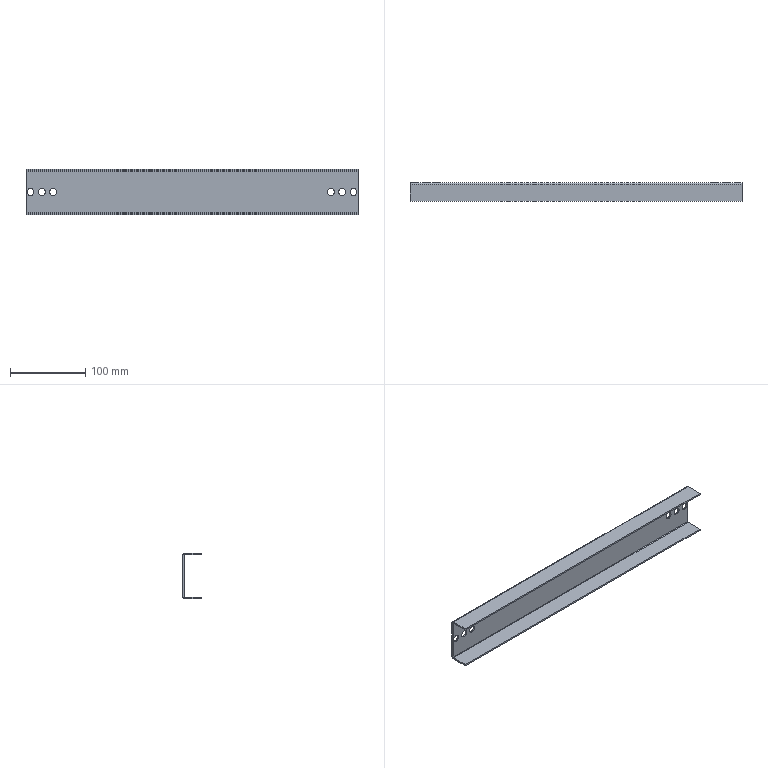Component | SolidWorks | 500CabinetWidthDoorCrossbeamAssembly-1_500CabinetWidthDoorCrossbeam-1 | 1 solid | 34 faces | box 440 x 25 x 60 mm | volume 91170 mm3 | plane 18 | cylinder 16 | commonest cylinder face diameters 9.2 x12 5.473 x2 1.473 x2 | material Plain Carbon Steel
STEP:
#1=COLOUR_RGB('',0.7922,0.8196,0.9333);
#2=FILL_AREA_STYLE_COLOUR('',#1);
#3=FILL_AREA_STYLE('',(#2));
#4=SURFACE_STYLE_FILL_AREA(#3);
#5=SURFACE_SIDE_STYLE('',(#4));
#6=SURFACE_STYLE_USAGE(.BOTH.,#5);
#7=PRESENTATION_STYLE_ASSIGNMENT((#6));
#8=CARTESIAN_POINT('',(-51.435,6.867,86.05));
#9=VERTEX_POINT('',#8);
#10=CARTESIAN_POINT('',(-51.435,6.867,86.412));
#11=VERTEX_POINT('',#10);
#12=CARTESIAN_POINT('',(-51.435,6.867,86.231));
#13=DIRECTION('',(-0.,1.,-0.));
#14=DIRECTION('',(0.,0.,1.));
#15=AXIS2_PLACEMENT_3D('',#12,#13,#14);
#16=CIRCLE('',#15,0.1811);
#17=EDGE_CURVE('',#9,#11,#16,.T.);
#18=ORIENTED_EDGE('',*,*,#17,.F.);
#19=CARTESIAN_POINT('',(-51.435,6.946,86.05));
#20=VERTEX_POINT('',#19);
#21=CARTESIAN_POINT('',(-51.435,6.867,86.05));
#22=DIRECTION('',(-0.,1.,-0.));
#23=VECTOR('',#22,39.37);
#24=LINE('',#21,#23);
#25=EDGE_CURVE('',#9,#20,#24,.T.);
#26=ORIENTED_EDGE('',*,*,#25,.T.);
#27=CARTESIAN_POINT('',(-51.435,6.946,86.412));
#28=VERTEX_POINT('',#27);
#29=CARTESIAN_POINT('',(-51.435,6.946,86.231));
#30=DIRECTION('',(-0.,1.,-0.));
#31=DIRECTION('',(0.,0.,1.));
#32=AXIS2_PLACEMENT_3D('',#29,#30,#31);
#33=CIRCLE('',#32,0.1811);
#34=EDGE_CURVE('',#20,#28,#33,.T.);
#35=ORIENTED_EDGE('',*,*,#34,.T.);
#36=CARTESIAN_POINT('',(-51.435,6.867,86.412));
#37=DIRECTION('',(-0.,1.,-0.));
#38=VECTOR('',#37,39.37);
#39=LINE('',#36,#38);
#40=EDGE_CURVE('',#11,#28,#39,.T.);
#41=ORIENTED_EDGE('',*,*,#40,.F.);
#42=EDGE_LOOP('',(#18,#26,#35,#41));
#43=FACE_OUTER_BOUND('',#42,.T.);
#44=CARTESIAN_POINT('',(-51.435,6.867,86.231));
#45=DIRECTION('',(-0.,1.,-0.));
#46=DIRECTION('',(0.,0.,1.));
#47=AXIS2_PLACEMENT_3D('',#44,#45,#46);
#48=CYLINDRICAL_SURFACE('',#47,0.1811);
#49=ADVANCED_FACE('',(#43),#48,.F.);
#50=CARTESIAN_POINT('',(-52.025,6.867,86.05));
#51=VERTEX_POINT('',#50);
#52=CARTESIAN_POINT('',(-52.025,6.867,86.412));
#53=VERTEX_POINT('',#52);
#54=CARTESIAN_POINT('',(-52.025,6.867,86.231));
#55=DIRECTION('',(-0.,1.,-0.));
#56=DIRECTION('',(0.,0.,1.));
#57=AXIS2_PLACEMENT_3D('',#54,#55,#56);
#58=CIRCLE('',#57,0.1811);
#59=EDGE_CURVE('',#51,#53,#58,.T.);
#60=ORIENTED_EDGE('',*,*,#59,.F.);
#61=CARTESIAN_POINT('',(-52.025,6.946,86.05));
#62=VERTEX_POINT('',#61);
#63=CARTESIAN_POINT('',(-52.025,6.867,86.05));
#64=DIRECTION('',(-0.,1.,-0.));
#65=VECTOR('',#64,39.37);
#66=LINE('',#63,#65);
#67=EDGE_CURVE('',#51,#62,#66,.T.);
#68=ORIENTED_EDGE('',*,*,#67,.T.);
#69=CARTESIAN_POINT('',(-52.025,6.946,86.412));
#70=VERTEX_POINT('',#69);
#71=CARTESIAN_POINT('',(-52.025,6.946,86.231));
#72=DIRECTION('',(-0.,1.,-0.));
#73=DIRECTION('',(0.,0.,1.));
#74=AXIS2_PLACEMENT_3D('',#71,#72,#73);
#75=CIRCLE('',#74,0.1811);
#76=EDGE_CURVE('',#62,#70,#75,.T.);
#77=ORIENTED_EDGE('',*,*,#76,.T.);
#78=CARTESIAN_POINT('',(-52.025,6.867,86.412));
#79=DIRECTION('',(-0.,1.,-0.));
#80=VECTOR('',#79,39.37);
#81=LINE('',#78,#80);
#82=EDGE_CURVE('',#53,#70,#81,.T.);
#83=ORIENTED_EDGE('',*,*,#82,.F.);
#84=EDGE_LOOP('',(#60,#68,#77,#83));
#85=FACE_OUTER_BOUND('',#84,.T.);
#86=CARTESIAN_POINT('',(-52.025,6.867,86.231));
#87=DIRECTION('',(-0.,1.,-0.));
#88=DIRECTION('',(0.,0.,1.));
#89=AXIS2_PLACEMENT_3D('',#86,#87,#88);
#90=CYLINDRICAL_SURFACE('',#89,0.1811);
#91=ADVANCED_FACE('',(#85),#90,.F.);
#92=CARTESIAN_POINT('',(-66.513,6.867,86.05));
#93=VERTEX_POINT('',#92);
#94=CARTESIAN_POINT('',(-66.513,6.867,86.412));
#95=VERTEX_POINT('',#94);
#96=CARTESIAN_POINT('',(-66.513,6.867,86.231));
#97=DIRECTION('',(-0.,1.,-0.));
#98=DIRECTION('',(0.,-0.,-1.));
#99=AXIS2_PLACEMENT_3D('',#96,#97,#98);
#100=CIRCLE('',#99,0.1811);
#101=EDGE_CURVE('',#93,#95,#100,.T.);
#102=ORIENTED_EDGE('',*,*,#101,.F.);
#103=CARTESIAN_POINT('',(-66.513,6.946,86.05));
#104=VERTEX_POINT('',#103);
#105=CARTESIAN_POINT('',(-66.513,6.867,86.05));
#106=DIRECTION('',(-0.,1.,-0.));
#107=VECTOR('',#106,39.37);
#108=LINE('',#105,#107);
#109=EDGE_CURVE('',#93,#104,#108,.T.);
#110=ORIENTED_EDGE('',*,*,#109,.T.);
#111=CARTESIAN_POINT('',(-66.513,6.946,86.412));
#112=VERTEX_POINT('',#111);
#113=CARTESIAN_POINT('',(-66.513,6.946,86.231));
#114=DIRECTION('',(-0.,1.,-0.));
#115=DIRECTION('',(0.,-0.,-1.));
#116=AXIS2_PLACEMENT_3D('',#113,#114,#115);
#117=CIRCLE('',#116,0.1811);
#118=EDGE_CURVE('',#104,#112,#117,.T.);
#119=ORIENTED_EDGE('',*,*,#118,.T.);
#120=CARTESIAN_POINT('',(-66.513,6.867,86.412));
#121=DIRECTION('',(-0.,1.,-0.));
#122=VECTOR('',#121,39.37);
#123=LINE('',#120,#122);
#124=EDGE_CURVE('',#95,#112,#123,.T.);
#125=ORIENTED_EDGE('',*,*,#124,.F.);
#126=EDGE_LOOP('',(#102,#110,#119,#125));
#127=FACE_OUTER_BOUND('',#126,.T.);
#128=CARTESIAN_POINT('',(-66.513,6.867,86.231));
#129=DIRECTION('',(-0.,1.,-0.));
#130=DIRECTION('',(0.,0.,1.));
#131=AXIS2_PLACEMENT_3D('',#128,#129,#130);
#132=CYLINDRICAL_SURFACE('',#131,0.1811);
#133=ADVANCED_FACE('',(#127),#132,.F.);
#134=CARTESIAN_POINT('',(-67.104,6.867,86.05));
#135=VERTEX_POINT('',#134);
#136=CARTESIAN_POINT('',(-67.104,6.867,86.412));
#137=VERTEX_POINT('',#136);
#138=CARTESIAN_POINT('',(-67.104,6.867,86.231));
#139=DIRECTION('',(-0.,1.,-0.));
#140=DIRECTION('',(0.,-0.,-1.));
#141=AXIS2_PLACEMENT_3D('',#138,#139,#140);
#142=CIRCLE('',#141,0.1811);
#143=EDGE_CURVE('',#135,#137,#142,.T.);
#144=ORIENTED_EDGE('',*,*,#143,.F.);
#145=CARTESIAN_POINT('',(-67.104,6.946,86.05));
#146=VERTEX_POINT('',#145);
#147=CARTESIAN_POINT('',(-67.104,6.867,86.05));
#148=DIRECTION('',(-0.,1.,-0.));
#149=VECTOR('',#148,39.37);
#150=LINE('',#147,#149);
#151=EDGE_CURVE('',#135,#146,#150,.T.);
#152=ORIENTED_EDGE('',*,*,#151,.T.);
#153=CARTESIAN_POINT('',(-67.104,6.946,86.412));
#154=VERTEX_POINT('',#153);
#155=CARTESIAN_POINT('',(-67.104,6.946,86.231));
#156=DIRECTION('',(-0.,1.,-0.));
#157=DIRECTION('',(0.,-0.,-1.));
#158=AXIS2_PLACEMENT_3D('',#155,#156,#157);
#159=CIRCLE('',#158,0.1811);
#160=EDGE_CURVE('',#146,#154,#159,.T.);
#161=ORIENTED_EDGE('',*,*,#160,.T.);
#162=CARTESIAN_POINT('',(-67.104,6.867,86.412));
#163=DIRECTION('',(-0.,1.,-0.));
#164=VECTOR('',#163,39.37);
#165=LINE('',#162,#164);
#166=EDGE_CURVE('',#137,#154,#165,.T.);
#167=ORIENTED_EDGE('',*,*,#166,.F.);
#168=EDGE_LOOP('',(#144,#152,#161,#167));
#169=FACE_OUTER_BOUND('',#168,.T.);
#170=CARTESIAN_POINT('',(-67.104,6.867,86.231));
#171=DIRECTION('',(-0.,1.,-0.));
#172=DIRECTION('',(0.,0.,1.));
#173=AXIS2_PLACEMENT_3D('',#170,#171,#172);
#174=CYLINDRICAL_SURFACE('',#173,0.1811);
#175=ADVANCED_FACE('',(#169),#174,.F.);
#176=CARTESIAN_POINT('',(-67.694,6.867,86.05));
#177=VERTEX_POINT('',#176);
#178=CARTESIAN_POINT('',(-67.694,6.867,86.412));
#179=VERTEX_POINT('',#178);
#180=CARTESIAN_POINT('',(-67.694,6.867,86.231));
#181=DIRECTION('',(-0.,1.,-0.));
#182=DIRECTION('',(0.,-0.,-1.));
#183=AXIS2_PLACEMENT_3D('',#180,#181,#182);
#184=CIRCLE('',#183,0.1811);
#185=EDGE_CURVE('',#177,#179,#184,.T.);
#186=ORIENTED_EDGE('',*,*,#185,.F.);
#187=CARTESIAN_POINT('',(-67.694,6.946,86.05));
#188=VERTEX_POINT('',#187);
#189=CARTESIAN_POINT('',(-67.694,6.867,86.05));
#190=DIRECTION('',(-0.,1.,-0.));
#191=VECTOR('',#190,39.37);
#192=LINE('',#189,#191);
#193=EDGE_CURVE('',#177,#188,#192,.T.);
#194=ORIENTED_EDGE('',*,*,#193,.T.);
#195=CARTESIAN_POINT('',(-67.694,6.946,86.412));
#196=VERTEX_POINT('',#195);
#197=CARTESIAN_POINT('',(-67.694,6.946,86.231));
#198=DIRECTION('',(-0.,1.,-0.));
#199=DIRECTION('',(0.,-0.,-1.));
#200=AXIS2_PLACEMENT_3D('',#197,#198,#199);
#201=CIRCLE('',#200,0.1811);
#202=EDGE_CURVE('',#188,#196,#201,.T.);
#203=ORIENTED_EDGE('',*,*,#202,.T.);
#204=CARTESIAN_POINT('',(-67.694,6.867,86.412));
#205=DIRECTION('',(-0.,1.,-0.));
#206=VECTOR('',#205,39.37);
#207=LINE('',#204,#206);
#208=EDGE_CURVE('',#179,#196,#207,.T.);
#209=ORIENTED_EDGE('',*,*,#208,.F.);
#210=EDGE_LOOP('',(#186,#194,#203,#209));
#211=FACE_OUTER_BOUND('',#210,.T.);
#212=CARTESIAN_POINT('',(-67.694,6.867,86.231));
#213=DIRECTION('',(-0.,1.,-0.));
#214=DIRECTION('',(0.,0.,1.));
#215=AXIS2_PLACEMENT_3D('',#212,#213,#214);
#216=CYLINDRICAL_SURFACE('',#215,0.1811);
#217=ADVANCED_FACE('',(#211),#216,.F.);
#218=CARTESIAN_POINT('',(-50.844,6.867,86.05));
#219=VERTEX_POINT('',#218);
#220=CARTESIAN_POINT('',(-50.844,6.867,86.412));
#221=VERTEX_POINT('',#220);
#222=CARTESIAN_POINT('',(-50.844,6.867,86.231));
#223=DIRECTION('',(-0.,1.,-0.));
#224=DIRECTION('',(0.,0.,1.));
#225=AXIS2_PLACEMENT_3D('',#222,#223,#224);
#226=CIRCLE('',#225,0.1811);
#227=EDGE_CURVE('',#219,#221,#226,.T.);
#228=ORIENTED_EDGE('',*,*,#227,.F.);
#229=CARTESIAN_POINT('',(-50.844,6.946,86.05));
#230=VERTEX_POINT('',#229);
#231=CARTESIAN_POINT('',(-50.844,6.867,86.05));
#232=DIRECTION('',(-0.,1.,-0.));
#233=VECTOR('',#232,39.37);
#234=LINE('',#231,#233);
#235=EDGE_CURVE('',#219,#230,#234,.T.);
#236=ORIENTED_EDGE('',*,*,#235,.T.);
#237=CARTESIAN_POINT('',(-50.844,6.946,86.412));
#238=VERTEX_POINT('',#237);
#239=CARTESIAN_POINT('',(-50.844,6.946,86.231));
#240=DIRECTION('',(-0.,1.,-0.));
#241=DIRECTION('',(0.,0.,1.));
#242=AXIS2_PLACEMENT_3D('',#239,#240,#241);
#243=CIRCLE('',#242,0.1811);
#244=EDGE_CURVE('',#230,#238,#243,.T.);
#245=ORIENTED_EDGE('',*,*,#244,.T.);
#246=CARTESIAN_POINT('',(-50.844,6.867,86.412));
#247=DIRECTION('',(-0.,1.,-0.));
#248=VECTOR('',#247,39.37);
#249=LINE('',#246,#248);
#250=EDGE_CURVE('',#221,#238,#249,.T.);
#251=ORIENTED_EDGE('',*,*,#250,.F.);
#252=EDGE_LOOP('',(#228,#236,#245,#251));
#253=FACE_OUTER_BOUND('',#252,.T.);
#254=CARTESIAN_POINT('',(-50.844,6.867,86.231));
#255=DIRECTION('',(-0.,1.,-0.));
#256=DIRECTION('',(0.,0.,1.));
#257=AXIS2_PLACEMENT_3D('',#254,#255,#256);
#258=CYLINDRICAL_SURFACE('',#257,0.1811);
#259=ADVANCED_FACE('',(#253),#258,.F.);
#260=CARTESIAN_POINT('',(-50.608,6.946,87.304));
#261=VERTEX_POINT('',#260);
#262=CARTESIAN_POINT('',(-50.608,6.867,87.304));
#263=VERTEX_POINT('',#262);
#264=CARTESIAN_POINT('',(-50.608,6.946,87.304));
#265=DIRECTION('',(0.,-1.,0.));
#266=VECTOR('',#265,39.37);
#267=LINE('',#264,#266);
#268=EDGE_CURVE('',#261,#263,#267,.T.);
#269=ORIENTED_EDGE('',*,*,#268,.F.);
#270=CARTESIAN_POINT('',(-50.608,6.838,87.412));
#271=VERTEX_POINT('',#270);
#272=CARTESIAN_POINT('',(-50.608,6.838,87.304));
#273=DIRECTION('',(-1.,-0.,-0.));
#274=DIRECTION('',(0.,0.,1.));
#275=AXIS2_PLACEMENT_3D('',#272,#273,#274);
#276=CIRCLE('',#275,0.1077);
#277=EDGE_CURVE('',#271,#261,#276,.T.);
#278=ORIENTED_EDGE('',*,*,#277,.F.);
#279=CARTESIAN_POINT('',(-50.608,6.838,87.333));
#280=VERTEX_POINT('',#279);
#281=CARTESIAN_POINT('',(-50.608,6.838,87.333));
#282=DIRECTION('',(-0.,0.,1.));
#283=VECTOR('',#282,39.37);
#284=LINE('',#281,#283);
#285=EDGE_CURVE('',#280,#271,#284,.T.);
#286=ORIENTED_EDGE('',*,*,#285,.F.);
#287=CARTESIAN_POINT('',(-50.608,6.838,87.304));
#288=DIRECTION('',(-1.,-0.,-0.));
#289=DIRECTION('',(0.,-1.,0.));
#290=AXIS2_PLACEMENT_3D('',#287,#288,#289);
#291=CIRCLE('',#290,0.029);
#292=EDGE_CURVE('',#280,#263,#291,.T.);
#293=ORIENTED_EDGE('',*,*,#292,.T.);
#294=EDGE_LOOP('',(#269,#278,#286,#293));
#295=FACE_OUTER_BOUND('',#294,.T.);
#296=CARTESIAN_POINT('',(-50.608,6.946,87.304));
#297=DIRECTION('',(1.,0.,0.));
#298=DIRECTION('',(-0.,0.,1.));
#299=AXIS2_PLACEMENT_3D('',#296,#297,#298);
#300=PLANE('',#299);
#301=ADVANCED_FACE('',(#295),#300,.T.);
#302=CARTESIAN_POINT('',(-50.608,6.946,85.158));
#303=VERTEX_POINT('',#302);
#304=CARTESIAN_POINT('',(-50.608,6.946,87.412));
#305=DIRECTION('',(0.,-0.,-1.));
#306=VECTOR('',#305,39.37);
#307=LINE('',#304,#306);
#308=EDGE_CURVE('',#261,#303,#307,.T.);
#309=ORIENTED_EDGE('',*,*,#308,.F.);
#310=ORIENTED_EDGE('',*,*,#268,.T.);
#311=CARTESIAN_POINT('',(-50.608,6.867,85.158));
#312=VERTEX_POINT('',#311);
#313=CARTESIAN_POINT('',(-50.608,6.867,87.412));
#314=DIRECTION('',(0.,-0.,-1.));
#315=VECTOR('',#314,39.37);
#316=LINE('',#313,#315);
#317=EDGE_CURVE('',#263,#312,#316,.T.);
#318=ORIENTED_EDGE('',*,*,#317,.T.);
#319=CARTESIAN_POINT('',(-50.608,6.867,85.158));
#320=DIRECTION('',(-0.,1.,-0.));
#321=VECTOR('',#320,39.37);
#322=LINE('',#319,#321);
#323=EDGE_CURVE('',#312,#303,#322,.T.);
#324=ORIENTED_EDGE('',*,*,#323,.T.);
#325=EDGE_LOOP('',(#309,#310,#318,#324));
#326=FACE_OUTER_BOUND('',#325,.T.);
#327=CARTESIAN_POINT('',(-50.608,6.838,87.333));
#328=DIRECTION('',(1.,0.,0.));
#329=DIRECTION('',(-0.,0.,1.));
#330=AXIS2_PLACEMENT_3D('',#327,#328,#329);
#331=PLANE('',#330);
#332=ADVANCED_FACE('',(#326),#331,.T.);
#333=CARTESIAN_POINT('',(-67.931,6.838,87.412));
#334=VERTEX_POINT('',#333);
#335=CARTESIAN_POINT('',(-67.931,6.838,87.333));
#336=VERTEX_POINT('',#335);
#337=CARTESIAN_POINT('',(-67.931,6.838,87.412));
#338=DIRECTION('',(0.,-0.,-1.));
#339=VECTOR('',#338,39.37);
#340=LINE('',#337,#339);
#341=EDGE_CURVE('',#334,#336,#340,.T.);
#342=ORIENTED_EDGE('',*,*,#341,.F.);
#343=CARTESIAN_POINT('',(-67.931,6.946,87.304));
#344=VERTEX_POINT('',#343);
#345=CARTESIAN_POINT('',(-67.931,6.838,87.304));
#346=DIRECTION('',(-1.,-0.,-0.));
#347=DIRECTION('',(0.,0.,1.));
#348=AXIS2_PLACEMENT_3D('',#345,#346,#347);
#349=CIRCLE('',#348,0.1077);
#350=EDGE_CURVE('',#334,#344,#349,.T.);
#351=ORIENTED_EDGE('',*,*,#350,.T.);
#352=CARTESIAN_POINT('',(-67.931,6.867,87.304));
#353=VERTEX_POINT('',#352);
#354=CARTESIAN_POINT('',(-67.931,6.867,87.304));
#355=DIRECTION('',(-0.,1.,-0.));
#356=VECTOR('',#355,39.37);
#357=LINE('',#354,#356);
#358=EDGE_CURVE('',#353,#344,#357,.T.);
#359=ORIENTED_EDGE('',*,*,#358,.F.);
#360=CARTESIAN_POINT('',(-67.931,6.838,87.304));
#361=DIRECTION('',(-1.,-0.,-0.));
#362=DIRECTION('',(0.,-1.,0.));
#363=AXIS2_PLACEMENT_3D('',#360,#361,#362);
#364=CIRCLE('',#363,0.029);
#365=EDGE_CURVE('',#336,#353,#364,.T.);
#366=ORIENTED_EDGE('',*,*,#365,.F.);
#367=EDGE_LOOP('',(#342,#351,#359,#366));
#368=FACE_OUTER_BOUND('',#367,.T.);
#369=CARTESIAN_POINT('',(-67.931,6.838,87.412));
#370=DIRECTION('',(-1.,-0.,-0.));
#371=DIRECTION('',(0.,-0.,-1.));
#372=AXIS2_PLACEMENT_3D('',#369,#370,#371);
#373=PLANE('',#372);
#374=ADVANCED_FACE('',(#368),#373,.T.);
#375=CARTESIAN_POINT('',(-67.931,5.961,87.412));
#376=VERTEX_POINT('',#375);
#377=CARTESIAN_POINT('',(-67.931,5.961,87.412));
#378=DIRECTION('',(-0.,1.,-0.));
#379=VECTOR('',#378,39.37);
#380=LINE('',#377,#379);
#381=EDGE_CURVE('',#376,#334,#380,.T.);
#382=ORIENTED_EDGE('',*,*,#381,.T.);
#383=ORIENTED_EDGE('',*,*,#341,.T.);
#384=CARTESIAN_POINT('',(-67.931,5.961,87.333));
#385=VERTEX_POINT('',#384);
#386=CARTESIAN_POINT('',(-67.931,5.961,87.333));
#387=DIRECTION('',(-0.,1.,-0.));
#388=VECTOR('',#387,39.37);
#389=LINE('',#386,#388);
#390=EDGE_CURVE('',#385,#336,#389,.T.);
#391=ORIENTED_EDGE('',*,*,#390,.F.);
#392=CARTESIAN_POINT('',(-67.931,5.961,87.333));
#393=DIRECTION('',(-0.,0.,1.));
#394=VECTOR('',#393,39.37);
#395=LINE('',#392,#394);
#396=EDGE_CURVE('',#385,#376,#395,.T.);
#397=ORIENTED_EDGE('',*,*,#396,.T.);
#398=EDGE_LOOP('',(#382,#383,#391,#397));
#399=FACE_OUTER_BOUND('',#398,.T.);
#400=CARTESIAN_POINT('',(-67.931,6.867,87.304));
#401=DIRECTION('',(-1.,-0.,-0.));
#402=DIRECTION('',(0.,-0.,-1.));
#403=AXIS2_PLACEMENT_3D('',#400,#401,#402);
#404=PLANE('',#403);
#405=ADVANCED_FACE('',(#399),#404,.T.);
#406=CARTESIAN_POINT('',(-50.608,6.838,85.05));
#407=VERTEX_POINT('',#406);
#408=CARTESIAN_POINT('',(-50.608,6.838,85.129));
#409=VERTEX_POINT('',#408);
#410=CARTESIAN_POINT('',(-50.608,6.838,85.05));
#411=DIRECTION('',(-0.,0.,1.));
#412=VECTOR('',#411,39.37);
#413=LINE('',#410,#412);
#414=EDGE_CURVE('',#407,#409,#413,.T.);
#415=ORIENTED_EDGE('',*,*,#414,.F.);
#416=CARTESIAN_POINT('',(-50.608,6.838,85.158));
#417=DIRECTION('',(-1.,-0.,-0.));
#418=DIRECTION('',(0.,0.,1.));
#419=AXIS2_PLACEMENT_3D('',#416,#417,#418);
#420=CIRCLE('',#419,0.1077);
#421=EDGE_CURVE('',#303,#407,#420,.T.);
#422=ORIENTED_EDGE('',*,*,#421,.F.);
#423=ORIENTED_EDGE('',*,*,#323,.F.);
#424=CARTESIAN_POINT('',(-50.608,6.838,85.158));
#425=DIRECTION('',(-1.,-0.,-0.));
#426=DIRECTION('',(0.,-1.,0.));
#427=AXIS2_PLACEMENT_3D('',#424,#425,#426);
#428=CIRCLE('',#427,0.029);
#429=EDGE_CURVE('',#312,#409,#428,.T.);
#430=ORIENTED_EDGE('',*,*,#429,.T.);
#431=EDGE_LOOP('',(#415,#422,#423,#430));
#432=FACE_OUTER_BOUND('',#431,.T.);
#433=CARTESIAN_POINT('',(-50.608,6.838,85.05));
#434=DIRECTION('',(1.,0.,0.));
#435=DIRECTION('',(-0.,0.,1.));
#436=AXIS2_PLACEMENT_3D('',#433,#434,#435);
#437=PLANE('',#436);
#438=ADVANCED_FACE('',(#432),#437,.T.);
#439=CARTESIAN_POINT('',(-50.608,5.961,85.05));
#440=VERTEX_POINT('',#439);
#441=CARTESIAN_POINT('',(-50.608,6.946,85.05));
#442=DIRECTION('',(0.,-1.,0.));
#443=VECTOR('',#442,39.37);
#444=LINE('',#441,#443);
#445=EDGE_CURVE('',#407,#440,#444,.T.);
#446=ORIENTED_EDGE('',*,*,#445,.F.);
#447=ORIENTED_EDGE('',*,*,#414,.T.);
#448=CARTESIAN_POINT('',(-50.608,5.961,85.129));
#449=VERTEX_POINT('',#448);
#450=CARTESIAN_POINT('',(-50.608,6.946,85.129));
#451=DIRECTION('',(0.,-1.,0.));
#452=VECTOR('',#451,39.37);
#453=LINE('',#450,#452);
#454=EDGE_CURVE('',#409,#449,#453,.T.);
#455=ORIENTED_EDGE('',*,*,#454,.T.);
#456=CARTESIAN_POINT('',(-50.608,5.961,85.05));
#457=DIRECTION('',(-0.,0.,1.));
#458=VECTOR('',#457,39.37);
#459=LINE('',#456,#458);
#460=EDGE_CURVE('',#440,#449,#459,.T.);
#461=ORIENTED_EDGE('',*,*,#460,.F.);
#462=EDGE_LOOP('',(#446,#447,#455,#461));
#463=FACE_OUTER_BOUND('',#462,.T.);
#464=CARTESIAN_POINT('',(-50.608,6.867,85.158));
#465=DIRECTION('',(1.,0.,0.));
#466=DIRECTION('',(-0.,0.,1.));
#467=AXIS2_PLACEMENT_3D('',#464,#465,#466);
#468=PLANE('',#467);
#469=ADVANCED_FACE('',(#463),#468,.T.);
#470=CARTESIAN_POINT('',(-67.931,6.946,85.158));
#471=VERTEX_POINT('',#470);
#472=CARTESIAN_POINT('',(-67.931,6.867,85.158));
#473=VERTEX_POINT('',#472);
#474=CARTESIAN_POINT('',(-67.931,6.946,85.158));
#475=DIRECTION('',(0.,-1.,0.));
#476=VECTOR('',#475,39.37);
#477=LINE('',#474,#476);
#478=EDGE_CURVE('',#471,#473,#477,.T.);
#479=ORIENTED_EDGE('',*,*,#478,.F.);
#480=CARTESIAN_POINT('',(-67.931,6.838,85.05));
#481=VERTEX_POINT('',#480);
#482=CARTESIAN_POINT('',(-67.931,6.838,85.158));
#483=DIRECTION('',(-1.,-0.,-0.));
#484=DIRECTION('',(0.,0.,1.));
#485=AXIS2_PLACEMENT_3D('',#482,#483,#484);
#486=CIRCLE('',#485,0.1077);
#487=EDGE_CURVE('',#471,#481,#486,.T.);
#488=ORIENTED_EDGE('',*,*,#487,.T.);
#489=CARTESIAN_POINT('',(-67.931,6.838,85.129));
#490=VERTEX_POINT('',#489);
#491=CARTESIAN_POINT('',(-67.931,6.838,85.129));
#492=DIRECTION('',(0.,-0.,-1.));
#493=VECTOR('',#492,39.37);
#494=LINE('',#491,#493);
#495=EDGE_CURVE('',#490,#481,#494,.T.);
#496=ORIENTED_EDGE('',*,*,#495,.F.);
#497=CARTESIAN_POINT('',(-67.931,6.838,85.158));
#498=DIRECTION('',(-1.,-0.,-0.));
#499=DIRECTION('',(0.,-1.,0.));
#500=AXIS2_PLACEMENT_3D('',#497,#498,#499);
#501=CIRCLE('',#500,0.029);
#502=EDGE_CURVE('',#473,#490,#501,.T.);
#503=ORIENTED_EDGE('',*,*,#502,.F.);
#504=EDGE_LOOP('',(#479,#488,#496,#503));
#505=FACE_OUTER_BOUND('',#504,.T.);
#506=CARTESIAN_POINT('',(-67.931,6.946,85.158));
#507=DIRECTION('',(-1.,-0.,-0.));
#508=DIRECTION('',(0.,-0.,-1.));
#509=AXIS2_PLACEMENT_3D('',#506,#507,#508);
#510=PLANE('',#509);
#511=ADVANCED_FACE('',(#505),#510,.T.);
#512=CARTESIAN_POINT('',(-67.931,6.946,87.412));
#513=DIRECTION('',(0.,-0.,-1.));
#514=VECTOR('',#513,39.37);
#515=LINE('',#512,#514);
#516=EDGE_CURVE('',#344,#471,#515,.T.);
#517=ORIENTED_EDGE('',*,*,#516,.T.);
#518=ORIENTED_EDGE('',*,*,#478,.T.);
#519=CARTESIAN_POINT('',(-67.931,6.867,87.412));
#520=DIRECTION('',(0.,-0.,-1.));
#521=VECTOR('',#520,39.37);
#522=LINE('',#519,#521);
#523=EDGE_CURVE('',#353,#473,#522,.T.);
#524=ORIENTED_EDGE('',*,*,#523,.F.);
#525=ORIENTED_EDGE('',*,*,#358,.T.);
#526=EDGE_LOOP('',(#517,#518,#524,#525));
#527=FACE_OUTER_BOUND('',#526,.T.);
#528=CARTESIAN_POINT('',(-67.931,6.838,85.129));
#529=DIRECTION('',(-1.,-0.,-0.));
#530=DIRECTION('',(0.,-0.,-1.));
#531=AXIS2_PLACEMENT_3D('',#528,#529,#530);
#532=PLANE('',#531);
#533=ADVANCED_FACE('',(#527),#532,.T.);
#534=CARTESIAN_POINT('',(-67.931,5.961,85.129));
#535=VERTEX_POINT('',#534);
#536=CARTESIAN_POINT('',(-67.931,6.946,85.129));
#537=DIRECTION('',(0.,-1.,0.));
#538=VECTOR('',#537,39.37);
#539=LINE('',#536,#538);
#540=EDGE_CURVE('',#490,#535,#539,.T.);
#541=ORIENTED_EDGE('',*,*,#540,.T.);
#542=CARTESIAN_POINT('',(-50.608,5.961,85.129));
#543=DIRECTION('',(-1.,-0.,-0.));
#544=VECTOR('',#543,39.37);
#545=LINE('',#542,#544);
#546=EDGE_CURVE('',#449,#535,#545,.T.);
#547=ORIENTED_EDGE('',*,*,#546,.F.);
#548=ORIENTED_EDGE('',*,*,#454,.F.);
#549=CARTESIAN_POINT('',(-50.608,6.838,85.129));
#550=DIRECTION('',(-1.,-0.,-0.));
#551=VECTOR('',#550,39.37);
#552=LINE('',#549,#551);
#553=EDGE_CURVE('',#409,#490,#552,.T.);
#554=ORIENTED_EDGE('',*,*,#553,.T.);
#555=EDGE_LOOP('',(#541,#547,#548,#554));
#556=FACE_OUTER_BOUND('',#555,.T.);
#557=CARTESIAN_POINT('',(-50.608,6.946,85.129));
#558=DIRECTION('',(0.,-0.,-1.));
#559=DIRECTION('',(-0.,1.,-0.));
#560=AXIS2_PLACEMENT_3D('',#557,#558,#559);
#561=PLANE('',#560);
#562=ADVANCED_FACE('',(#556),#561,.F.);
#563=CARTESIAN_POINT('',(-67.931,5.961,85.05));
#564=VERTEX_POINT('',#563);
#565=CARTESIAN_POINT('',(-67.931,5.961,85.05));
#566=DIRECTION('',(-0.,0.,1.));
#567=VECTOR('',#566,39.37);
#568=LINE('',#565,#567);
#569=EDGE_CURVE('',#564,#535,#568,.T.);
#570=ORIENTED_EDGE('',*,*,#569,.F.);
#571=CARTESIAN_POINT('',(-50.608,5.961,85.05));
#572=DIRECTION('',(-1.,-0.,-0.));
#573=VECTOR('',#572,39.37);
#574=LINE('',#571,#573);
#575=EDGE_CURVE('',#440,#564,#574,.T.);
#576=ORIENTED_EDGE('',*,*,#575,.F.);
#577=ORIENTED_EDGE('',*,*,#460,.T.);
#578=ORIENTED_EDGE('',*,*,#546,.T.);
#579=EDGE_LOOP('',(#570,#576,#577,#578));
#580=FACE_OUTER_BOUND('',#579,.T.);
#581=CARTESIAN_POINT('',(-50.608,5.961,85.05));
#582=DIRECTION('',(0.,-1.,0.));
#583=DIRECTION('',(0.,-0.,-1.));
#584=AXIS2_PLACEMENT_3D('',#581,#582,#583);
#585=PLANE('',#584);
#586=ADVANCED_FACE('',(#580),#585,.T.);
#587=CARTESIAN_POINT('',(-67.931,6.946,85.05));
#588=DIRECTION('',(0.,-1.,0.));
#589=VECTOR('',#588,39.37);
#590=LINE('',#587,#589);
#591=EDGE_CURVE('',#481,#564,#590,.T.);
#592=ORIENTED_EDGE('',*,*,#591,.F.);
#593=CARTESIAN_POINT('',(-50.608,6.838,85.05));
#594=DIRECTION('',(-1.,-0.,-0.));
#595=VECTOR('',#594,39.37);
#596=LINE('',#593,#595);
#597=EDGE_CURVE('',#407,#481,#596,.T.);
#598=ORIENTED_EDGE('',*,*,#597,.F.);
#599=ORIENTED_EDGE('',*,*,#445,.T.);
#600=ORIENTED_EDGE('',*,*,#575,.T.);
#601=EDGE_LOOP('',(#592,#598,#599,#600));
#602=FACE_OUTER_BOUND('',#601,.T.);
#603=CARTESIAN_POINT('',(-50.608,6.946,85.05));
#604=DIRECTION('',(0.,-0.,-1.));
#605=DIRECTION('',(-0.,1.,-0.));
#606=AXIS2_PLACEMENT_3D('',#603,#604,#605);
#607=PLANE('',#606);
#608=ADVANCED_FACE('',(#602),#607,.T.);
#609=ORIENTED_EDGE('',*,*,#487,.F.);
#610=CARTESIAN_POINT('',(-50.608,6.946,85.158));
#611=DIRECTION('',(-1.,-0.,-0.));
#612=VECTOR('',#611,39.37);
#613=LINE('',#610,#612);
#614=EDGE_CURVE('',#303,#471,#613,.T.);
#615=ORIENTED_EDGE('',*,*,#614,.F.);
#616=ORIENTED_EDGE('',*,*,#421,.T.);
#617=ORIENTED_EDGE('',*,*,#597,.T.);
#618=EDGE_LOOP('',(#609,#615,#616,#617));
#619=FACE_OUTER_BOUND('',#618,.T.);
#620=CARTESIAN_POINT('',(-50.608,6.838,85.158));
#621=DIRECTION('',(-1.,-0.,-0.));
#622=DIRECTION('',(0.,-0.,-1.));
#623=AXIS2_PLACEMENT_3D('',#620,#621,#622);
#624=CYLINDRICAL_SURFACE('',#623,0.1077);
#625=ADVANCED_FACE('',(#619),#624,.T.);
#626=CARTESIAN_POINT('',(-51.435,6.946,86.231));
#627=DIRECTION('',(-0.,1.,-0.));
#628=DIRECTION('',(0.,0.,1.));
#629=AXIS2_PLACEMENT_3D('',#626,#627,#628);
#630=CIRCLE('',#629,0.1811);
#631=EDGE_CURVE('',#28,#20,#630,.T.);
#632=ORIENTED_EDGE('',*,*,#631,.F.);
#633=ORIENTED_EDGE('',*,*,#34,.F.);
#634=EDGE_LOOP('',(#632,#633));
#635=FACE_BOUND('',#634,.T.);
#636=CARTESIAN_POINT('',(-52.025,6.946,86.231));
#637=DIRECTION('',(-0.,1.,-0.));
#638=DIRECTION('',(0.,0.,1.));
#639=AXIS2_PLACEMENT_3D('',#636,#637,#638);
#640=CIRCLE('',#639,0.1811);
#641=EDGE_CURVE('',#70,#62,#640,.T.);
#642=ORIENTED_EDGE('',*,*,#641,.F.);
#643=ORIENTED_EDGE('',*,*,#76,.F.);
#644=EDGE_LOOP('',(#642,#643));
#645=FACE_BOUND('',#644,.T.);
#646=CARTESIAN_POINT('',(-66.513,6.946,86.231));
#647=DIRECTION('',(-0.,1.,-0.));
#648=DIRECTION('',(0.,-0.,-1.));
#649=AXIS2_PLACEMENT_3D('',#646,#647,#648);
#650=CIRCLE('',#649,0.1811);
#651=EDGE_CURVE('',#112,#104,#650,.T.);
#652=ORIENTED_EDGE('',*,*,#651,.F.);
#653=ORIENTED_EDGE('',*,*,#118,.F.);
#654=EDGE_LOOP('',(#652,#653));
#655=FACE_BOUND('',#654,.T.);
#656=CARTESIAN_POINT('',(-67.104,6.946,86.231));
#657=DIRECTION('',(-0.,1.,-0.));
#658=DIRECTION('',(0.,-0.,-1.));
#659=AXIS2_PLACEMENT_3D('',#656,#657,#658);
#660=CIRCLE('',#659,0.1811);
#661=EDGE_CURVE('',#154,#146,#660,.T.);
#662=ORIENTED_EDGE('',*,*,#661,.F.);
#663=ORIENTED_EDGE('',*,*,#160,.F.);
#664=EDGE_LOOP('',(#662,#663));
#665=FACE_BOUND('',#664,.T.);
#666=CARTESIAN_POINT('',(-67.694,6.946,86.231));
#667=DIRECTION('',(-0.,1.,-0.));
#668=DIRECTION('',(0.,-0.,-1.));
#669=AXIS2_PLACEMENT_3D('',#666,#667,#668);
#670=CIRCLE('',#669,0.1811);
#671=EDGE_CURVE('',#196,#188,#670,.T.);
#672=ORIENTED_EDGE('',*,*,#671,.F.);
#673=ORIENTED_EDGE('',*,*,#202,.F.);
#674=EDGE_LOOP('',(#672,#673));
#675=FACE_BOUND('',#674,.T.);
#676=CARTESIAN_POINT('',(-50.844,6.946,86.231));
#677=DIRECTION('',(-0.,1.,-0.));
#678=DIRECTION('',(0.,0.,1.));
#679=AXIS2_PLACEMENT_3D('',#676,#677,#678);
#680=CIRCLE('',#679,0.1811);
#681=EDGE_CURVE('',#238,#230,#680,.T.);
#682=ORIENTED_EDGE('',*,*,#681,.F.);
#683=ORIENTED_EDGE('',*,*,#244,.F.);
#684=EDGE_LOOP('',(#682,#683));
#685=FACE_BOUND('',#684,.T.);
#686=ORIENTED_EDGE('',*,*,#516,.F.);
#687=CARTESIAN_POINT('',(-50.608,6.946,87.304));
#688=DIRECTION('',(-1.,-0.,-0.));
#689=VECTOR('',#688,39.37);
#690=LINE('',#687,#689);
#691=EDGE_CURVE('',#261,#344,#690,.T.);
#692=ORIENTED_EDGE('',*,*,#691,.F.);
#693=ORIENTED_EDGE('',*,*,#308,.T.);
#694=ORIENTED_EDGE('',*,*,#614,.T.);
#695=EDGE_LOOP('',(#686,#692,#693,#694));
#696=FACE_OUTER_BOUND('',#695,.T.);
#697=CARTESIAN_POINT('',(-50.608,6.946,87.412));
#698=DIRECTION('',(-0.,1.,-0.));
#699=DIRECTION('',(-0.,0.,1.));
#700=AXIS2_PLACEMENT_3D('',#697,#698,#699);
#701=PLANE('',#700);
#702=ADVANCED_FACE('',(#635,#645,#655,#665,#675,#685,#696),#701,.T.);
#703=ORIENTED_EDGE('',*,*,#350,.F.);
#704=CARTESIAN_POINT('',(-50.608,6.838,87.412));
#705=DIRECTION('',(-1.,-0.,-0.));
#706=VECTOR('',#705,39.37);
#707=LINE('',#704,#706);
#708=EDGE_CURVE('',#271,#334,#707,.T.);
#709=ORIENTED_EDGE('',*,*,#708,.F.);
#710=ORIENTED_EDGE('',*,*,#277,.T.);
#711=ORIENTED_EDGE('',*,*,#691,.T.);
#712=EDGE_LOOP('',(#703,#709,#710,#711));
#713=FACE_OUTER_BOUND('',#712,.T.);
#714=CARTESIAN_POINT('',(-50.608,6.838,87.304));
#715=DIRECTION('',(-1.,-0.,-0.));
#716=DIRECTION('',(0.,-0.,-1.));
#717=AXIS2_PLACEMENT_3D('',#714,#715,#716);
#718=CYLINDRICAL_SURFACE('',#717,0.1077);
#719=ADVANCED_FACE('',(#713),#718,.T.);
#720=ORIENTED_EDGE('',*,*,#381,.F.);
#721=CARTESIAN_POINT('',(-50.608,5.961,87.412));
#722=VERTEX_POINT('',#721);
#723=CARTESIAN_POINT('',(-50.608,5.961,87.412));
#724=DIRECTION('',(-1.,-0.,-0.));
#725=VECTOR('',#724,39.37);
#726=LINE('',#723,#725);
#727=EDGE_CURVE('',#722,#376,#726,.T.);
#728=ORIENTED_EDGE('',*,*,#727,.F.);
#729=CARTESIAN_POINT('',(-50.608,5.961,87.412));
#730=DIRECTION('',(-0.,1.,-0.));
#731=VECTOR('',#730,39.37);
#732=LINE('',#729,#731);
#733=EDGE_CURVE('',#722,#271,#732,.T.);
#734=ORIENTED_EDGE('',*,*,#733,.T.);
#735=ORIENTED_EDGE('',*,*,#708,.T.);
#736=EDGE_LOOP('',(#720,#728,#734,#735));
#737=FACE_OUTER_BOUND('',#736,.T.);
#738=CARTESIAN_POINT('',(-50.608,5.961,87.412));
#739=DIRECTION('',(-0.,0.,1.));
#740=DIRECTION('',(0.,-1.,0.));
#741=AXIS2_PLACEMENT_3D('',#738,#739,#740);
#742=PLANE('',#741);
#743=ADVANCED_FACE('',(#737),#742,.T.);
#744=ORIENTED_EDGE('',*,*,#396,.F.);
#745=CARTESIAN_POINT('',(-50.608,5.961,87.333));
#746=VERTEX_POINT('',#745);
#747=CARTESIAN_POINT('',(-50.608,5.961,87.333));
#748=DIRECTION('',(-1.,-0.,-0.));
#749=VECTOR('',#748,39.37);
#750=LINE('',#747,#749);
#751=EDGE_CURVE('',#746,#385,#750,.T.);
#752=ORIENTED_EDGE('',*,*,#751,.F.);
#753=CARTESIAN_POINT('',(-50.608,5.961,87.333));
#754=DIRECTION('',(-0.,0.,1.));
#755=VECTOR('',#754,39.37);
#756=LINE('',#753,#755);
#757=EDGE_CURVE('',#746,#722,#756,.T.);
#758=ORIENTED_EDGE('',*,*,#757,.T.);
#759=ORIENTED_EDGE('',*,*,#727,.T.);
#760=EDGE_LOOP('',(#744,#752,#758,#759));
#761=FACE_OUTER_BOUND('',#760,.T.);
#762=CARTESIAN_POINT('',(-50.608,5.961,87.333));
#763=DIRECTION('',(0.,-1.,0.));
#764=DIRECTION('',(0.,-0.,-1.));
#765=AXIS2_PLACEMENT_3D('',#762,#763,#764);
#766=PLANE('',#765);
#767=ADVANCED_FACE('',(#761),#766,.T.);
#768=ORIENTED_EDGE('',*,*,#390,.T.);
#769=CARTESIAN_POINT('',(-50.608,6.838,87.333));
#770=DIRECTION('',(-1.,-0.,-0.));
#771=VECTOR('',#770,39.37);
#772=LINE('',#769,#771);
#773=EDGE_CURVE('',#280,#336,#772,.T.);
#774=ORIENTED_EDGE('',*,*,#773,.F.);
#775=CARTESIAN_POINT('',(-50.608,5.961,87.333));
#776=DIRECTION('',(-0.,1.,-0.));
#777=VECTOR('',#776,39.37);
#778=LINE('',#775,#777);
#779=EDGE_CURVE('',#746,#280,#778,.T.);
#780=ORIENTED_EDGE('',*,*,#779,.F.);
#781=ORIENTED_EDGE('',*,*,#751,.T.);
#782=EDGE_LOOP('',(#768,#774,#780,#781));
#783=FACE_OUTER_BOUND('',#782,.T.);
#784=CARTESIAN_POINT('',(-50.608,5.961,87.333));
#785=DIRECTION('',(-0.,0.,1.));
#786=DIRECTION('',(0.,-1.,0.));
#787=AXIS2_PLACEMENT_3D('',#784,#785,#786);
#788=PLANE('',#787);
#789=ADVANCED_FACE('',(#783),#788,.F.);
#790=ORIENTED_EDGE('',*,*,#365,.T.);
#791=CARTESIAN_POINT('',(-50.608,6.867,87.304));
#792=DIRECTION('',(-1.,-0.,-0.));
#793=VECTOR('',#792,39.37);
#794=LINE('',#791,#793);
#795=EDGE_CURVE('',#263,#353,#794,.T.);
#796=ORIENTED_EDGE('',*,*,#795,.F.);
#797=ORIENTED_EDGE('',*,*,#292,.F.);
#798=ORIENTED_EDGE('',*,*,#773,.T.);
#799=EDGE_LOOP('',(#790,#796,#797,#798));
#800=FACE_OUTER_BOUND('',#799,.T.);
#801=CARTESIAN_POINT('',(-50.608,6.838,87.304));
#802=DIRECTION('',(-1.,-0.,-0.));
#803=DIRECTION('',(0.,0.,-1.));
#804=AXIS2_PLACEMENT_3D('',#801,#802,#803);
#805=CYLINDRICAL_SURFACE('',#804,0.029);
#806=ADVANCED_FACE('',(#800),#805,.F.);
#807=CARTESIAN_POINT('',(-51.435,6.867,86.231));
#808=DIRECTION('',(-0.,1.,-0.));
#809=DIRECTION('',(0.,0.,1.));
#810=AXIS2_PLACEMENT_3D('',#807,#808,#809);
#811=CIRCLE('',#810,0.1811);
#812=EDGE_CURVE('',#11,#9,#811,.T.);
#813=ORIENTED_EDGE('',*,*,#812,.T.);
#814=ORIENTED_EDGE('',*,*,#17,.T.);
#815=EDGE_LOOP('',(#813,#814));
#816=FACE_BOUND('',#815,.T.);
#817=CARTESIAN_POINT('',(-52.025,6.867,86.231));
#818=DIRECTION('',(-0.,1.,-0.));
#819=DIRECTION('',(0.,0.,1.));
#820=AXIS2_PLACEMENT_3D('',#817,#818,#819);
#821=CIRCLE('',#820,0.1811);
#822=EDGE_CURVE('',#53,#51,#821,.T.);
#823=ORIENTED_EDGE('',*,*,#822,.T.);
#824=ORIENTED_EDGE('',*,*,#59,.T.);
#825=EDGE_LOOP('',(#823,#824));
#826=FACE_BOUND('',#825,.T.);
#827=CARTESIAN_POINT('',(-66.513,6.867,86.231));
#828=DIRECTION('',(-0.,1.,-0.));
#829=DIRECTION('',(0.,-0.,-1.));
#830=AXIS2_PLACEMENT_3D('',#827,#828,#829);
#831=CIRCLE('',#830,0.1811);
#832=EDGE_CURVE('',#95,#93,#831,.T.);
#833=ORIENTED_EDGE('',*,*,#832,.T.);
#834=ORIENTED_EDGE('',*,*,#101,.T.);
#835=EDGE_LOOP('',(#833,#834));
#836=FACE_BOUND('',#835,.T.);
#837=CARTESIAN_POINT('',(-67.104,6.867,86.231));
#838=DIRECTION('',(-0.,1.,-0.));
#839=DIRECTION('',(0.,-0.,-1.));
#840=AXIS2_PLACEMENT_3D('',#837,#838,#839);
#841=CIRCLE('',#840,0.1811);
#842=EDGE_CURVE('',#137,#135,#841,.T.);
#843=ORIENTED_EDGE('',*,*,#842,.T.);
#844=ORIENTED_EDGE('',*,*,#143,.T.);
#845=EDGE_LOOP('',(#843,#844));
#846=FACE_BOUND('',#845,.T.);
#847=CARTESIAN_POINT('',(-67.694,6.867,86.231));
#848=DIRECTION('',(-0.,1.,-0.));
#849=DIRECTION('',(0.,-0.,-1.));
#850=AXIS2_PLACEMENT_3D('',#847,#848,#849);
#851=CIRCLE('',#850,0.1811);
#852=EDGE_CURVE('',#179,#177,#851,.T.);
#853=ORIENTED_EDGE('',*,*,#852,.T.);
#854=ORIENTED_EDGE('',*,*,#185,.T.);
#855=EDGE_LOOP('',(#853,#854));
#856=FACE_BOUND('',#855,.T.);
#857=CARTESIAN_POINT('',(-50.844,6.867,86.231));
#858=DIRECTION('',(-0.,1.,-0.));
#859=DIRECTION('',(0.,0.,1.));
#860=AXIS2_PLACEMENT_3D('',#857,#858,#859);
#861=CIRCLE('',#860,0.1811);
#862=EDGE_CURVE('',#221,#219,#861,.T.);
#863=ORIENTED_EDGE('',*,*,#862,.T.);
#864=ORIENTED_EDGE('',*,*,#227,.T.);
#865=EDGE_LOOP('',(#863,#864));
#866=FACE_BOUND('',#865,.T.);
#867=ORIENTED_EDGE('',*,*,#523,.T.);
#868=CARTESIAN_POINT('',(-50.608,6.867,85.158));
#869=DIRECTION('',(-1.,-0.,-0.));
#870=VECTOR('',#869,39.37);
#871=LINE('',#868,#870);
#872=EDGE_CURVE('',#312,#473,#871,.T.);
#873=ORIENTED_EDGE('',*,*,#872,.F.);
#874=ORIENTED_EDGE('',*,*,#317,.F.);
#875=ORIENTED_EDGE('',*,*,#795,.T.);
#876=EDGE_LOOP('',(#867,#873,#874,#875));
#877=FACE_OUTER_BOUND('',#876,.T.);
#878=CARTESIAN_POINT('',(-50.608,6.867,87.412));
#879=DIRECTION('',(-0.,1.,-0.));
#880=DIRECTION('',(-0.,0.,1.));
#881=AXIS2_PLACEMENT_3D('',#878,#879,#880);
#882=PLANE('',#881);
#883=ADVANCED_FACE('',(#816,#826,#836,#846,#856,#866,#877),#882,.F.);
#884=ORIENTED_EDGE('',*,*,#502,.T.);
#885=ORIENTED_EDGE('',*,*,#553,.F.);
#886=ORIENTED_EDGE('',*,*,#429,.F.);
#887=ORIENTED_EDGE('',*,*,#872,.T.);
#888=EDGE_LOOP('',(#884,#885,#886,#887));
#889=FACE_OUTER_BOUND('',#888,.T.);
#890=CARTESIAN_POINT('',(-50.608,6.838,85.158));
#891=DIRECTION('',(-1.,-0.,-0.));
#892=DIRECTION('',(0.,0.,-1.));
#893=AXIS2_PLACEMENT_3D('',#890,#891,#892);
#894=CYLINDRICAL_SURFACE('',#893,0.029);
#895=ADVANCED_FACE('',(#889),#894,.F.);
#896=ORIENTED_EDGE('',*,*,#779,.T.);
#897=ORIENTED_EDGE('',*,*,#285,.T.);
#898=ORIENTED_EDGE('',*,*,#733,.F.);
#899=ORIENTED_EDGE('',*,*,#757,.F.);
#900=EDGE_LOOP('',(#896,#897,#898,#899));
#901=FACE_OUTER_BOUND('',#900,.T.);
#902=CARTESIAN_POINT('',(-50.608,6.838,85.158));
#903=DIRECTION('',(1.,0.,0.));
#904=DIRECTION('',(0.,-1.,0.));
#905=AXIS2_PLACEMENT_3D('',#902,#903,#904);
#906=PLANE('',#905);
#907=ADVANCED_FACE('',(#901),#906,.T.);
#908=ORIENTED_EDGE('',*,*,#540,.F.);
#909=ORIENTED_EDGE('',*,*,#495,.T.);
#910=ORIENTED_EDGE('',*,*,#591,.T.);
#911=ORIENTED_EDGE('',*,*,#569,.T.);
#912=EDGE_LOOP('',(#908,#909,#910,#911));
#913=FACE_OUTER_BOUND('',#912,.T.);
#914=CARTESIAN_POINT('',(-67.931,6.838,85.158));
#915=DIRECTION('',(1.,0.,0.));
#916=DIRECTION('',(0.,-1.,0.));
#917=AXIS2_PLACEMENT_3D('',#914,#915,#916);
#918=PLANE('',#917);
#919=ADVANCED_FACE('',(#913),#918,.F.);
#920=ORIENTED_EDGE('',*,*,#235,.F.);
#921=ORIENTED_EDGE('',*,*,#862,.F.);
#922=ORIENTED_EDGE('',*,*,#250,.T.);
#923=ORIENTED_EDGE('',*,*,#681,.T.);
#924=EDGE_LOOP('',(#920,#921,#922,#923));
#925=FACE_OUTER_BOUND('',#924,.T.);
#926=CARTESIAN_POINT('',(-50.844,6.867,86.231));
#927=DIRECTION('',(-0.,1.,-0.));
#928=DIRECTION('',(0.,0.,1.));
#929=AXIS2_PLACEMENT_3D('',#926,#927,#928);
#930=CYLINDRICAL_SURFACE('',#929,0.1811);
#931=ADVANCED_FACE('',(#925),#930,.F.);
#932=ORIENTED_EDGE('',*,*,#193,.F.);
#933=ORIENTED_EDGE('',*,*,#852,.F.);
#934=ORIENTED_EDGE('',*,*,#208,.T.);
#935=ORIENTED_EDGE('',*,*,#671,.T.);
#936=EDGE_LOOP('',(#932,#933,#934,#935));
#937=FACE_OUTER_BOUND('',#936,.T.);
#938=CARTESIAN_POINT('',(-67.694,6.867,86.231));
#939=DIRECTION('',(-0.,1.,-0.));
#940=DIRECTION('',(0.,0.,1.));
#941=AXIS2_PLACEMENT_3D('',#938,#939,#940);
#942=CYLINDRICAL_SURFACE('',#941,0.1811);
#943=ADVANCED_FACE('',(#937),#942,.F.);
#944=ORIENTED_EDGE('',*,*,#151,.F.);
#945=ORIENTED_EDGE('',*,*,#842,.F.);
#946=ORIENTED_EDGE('',*,*,#166,.T.);
#947=ORIENTED_EDGE('',*,*,#661,.T.);
#948=EDGE_LOOP('',(#944,#945,#946,#947));
#949=FACE_OUTER_BOUND('',#948,.T.);
#950=CARTESIAN_POINT('',(-67.104,6.867,86.231));
#951=DIRECTION('',(-0.,1.,-0.));
#952=DIRECTION('',(0.,0.,1.));
#953=AXIS2_PLACEMENT_3D('',#950,#951,#952);
#954=CYLINDRICAL_SURFACE('',#953,0.1811);
#955=ADVANCED_FACE('',(#949),#954,.F.);
#956=ORIENTED_EDGE('',*,*,#109,.F.);
#957=ORIENTED_EDGE('',*,*,#832,.F.);
#958=ORIENTED_EDGE('',*,*,#124,.T.);
#959=ORIENTED_EDGE('',*,*,#651,.T.);
#960=EDGE_LOOP('',(#956,#957,#958,#959));
#961=FACE_OUTER_BOUND('',#960,.T.);
#962=CARTESIAN_POINT('',(-66.513,6.867,86.231));
#963=DIRECTION('',(-0.,1.,-0.));
#964=DIRECTION('',(0.,0.,1.));
#965=AXIS2_PLACEMENT_3D('',#962,#963,#964);
#966=CYLINDRICAL_SURFACE('',#965,0.1811);
#967=ADVANCED_FACE('',(#961),#966,.F.);
#968=ORIENTED_EDGE('',*,*,#67,.F.);
#969=ORIENTED_EDGE('',*,*,#822,.F.);
#970=ORIENTED_EDGE('',*,*,#82,.T.);
#971=ORIENTED_EDGE('',*,*,#641,.T.);
#972=EDGE_LOOP('',(#968,#969,#970,#971));
#973=FACE_OUTER_BOUND('',#972,.T.);
#974=CARTESIAN_POINT('',(-52.025,6.867,86.231));
#975=DIRECTION('',(-0.,1.,-0.));
#976=DIRECTION('',(0.,0.,1.));
#977=AXIS2_PLACEMENT_3D('',#974,#975,#976);
#978=CYLINDRICAL_SURFACE('',#977,0.1811);
#979=ADVANCED_FACE('',(#973),#978,.F.);
#980=ORIENTED_EDGE('',*,*,#25,.F.);
#981=ORIENTED_EDGE('',*,*,#812,.F.);
#982=ORIENTED_EDGE('',*,*,#40,.T.);
#983=ORIENTED_EDGE('',*,*,#631,.T.);
#984=EDGE_LOOP('',(#980,#981,#982,#983));
#985=FACE_OUTER_BOUND('',#984,.T.);
#986=CARTESIAN_POINT('',(-51.435,6.867,86.231));
#987=DIRECTION('',(-0.,1.,-0.));
#988=DIRECTION('',(0.,0.,1.));
#989=AXIS2_PLACEMENT_3D('',#986,#987,#988);
#990=CYLINDRICAL_SURFACE('',#989,0.1811);
#991=ADVANCED_FACE('',(#985),#990,.F.);
#992=CLOSED_SHELL('',(#49,#91,#133,#175,#217,#259,#301,#332,#374,#405,#438,#469,#511,#533,#562,#586,#608,#625,#702,#719,#743,#767,#789,#806,#883,#895,#907,#919,#931,#943,#955,#967,#979,#991));
#993=MANIFOLD_SOLID_BREP('',#992);
#994=STYLED_ITEM('',(#7),#993);
#995=PRESENTATION_LAYER_ASSIGNMENT('','',(#994));
#996=(LENGTH_UNIT()NAMED_UNIT(*)SI_UNIT($,.METRE.));
#997=LENGTH_MEASURE_WITH_UNIT(LENGTH_MEASURE(0.0254),#996);
#998=DIMENSIONAL_EXPONENTS(1.,0.,0.,0.,0.,0.,0.);
#999=(CONVERSION_BASED_UNIT('',#997)LENGTH_UNIT()NAMED_UNIT(#998));
#1000=UNCERTAINTY_MEASURE_WITH_UNIT(LENGTH_MEASURE(0.00001),#999,'','');
#1001=(NAMED_UNIT(*)PLANE_ANGLE_UNIT()SI_UNIT($,.RADIAN.));
#1002=(NAMED_UNIT(*)SI_UNIT($,.STERADIAN.)SOLID_ANGLE_UNIT());
#1003=(GEOMETRIC_REPRESENTATION_CONTEXT(3)GLOBAL_UNCERTAINTY_ASSIGNED_CONTEXT((#1000))GLOBAL_UNIT_ASSIGNED_CONTEXT((#999,#1001,#1002))REPRESENTATION_CONTEXT('',''));
#1004=MECHANICAL_DESIGN_GEOMETRIC_PRESENTATION_REPRESENTATION('',(#994),#1003);
#1005=CARTESIAN_POINT('',(0.,0.,0.));
#1006=DIRECTION('',(0.,0.,1.));
#1007=DIRECTION('',(1.,0.,0.));
#1008=AXIS2_PLACEMENT_3D('',#1005,#1006,#1007);
#1009=(LENGTH_UNIT()NAMED_UNIT(*)SI_UNIT($,.METRE.));
#1010=LENGTH_MEASURE_WITH_UNIT(LENGTH_MEASURE(0.0254),#1009);
#1011=DIMENSIONAL_EXPONENTS(1.,0.,0.,0.,0.,0.,0.);
#1012=(CONVERSION_BASED_UNIT('',#1010)LENGTH_UNIT()NAMED_UNIT(#1011));
#1013=UNCERTAINTY_MEASURE_WITH_UNIT(LENGTH_MEASURE(0.00001),#1012,'','');
#1014=(NAMED_UNIT(*)PLANE_ANGLE_UNIT()SI_UNIT($,.RADIAN.));
#1015=(NAMED_UNIT(*)SI_UNIT($,.STERADIAN.)SOLID_ANGLE_UNIT());
#1016=(GEOMETRIC_REPRESENTATION_CONTEXT(3)GLOBAL_UNCERTAINTY_ASSIGNED_CONTEXT((#1013))GLOBAL_UNIT_ASSIGNED_CONTEXT((#1012,#1014,#1015))REPRESENTATION_CONTEXT('',''));
#1017=ADVANCED_BREP_SHAPE_REPRESENTATION('',(#993,#1008),#1016);